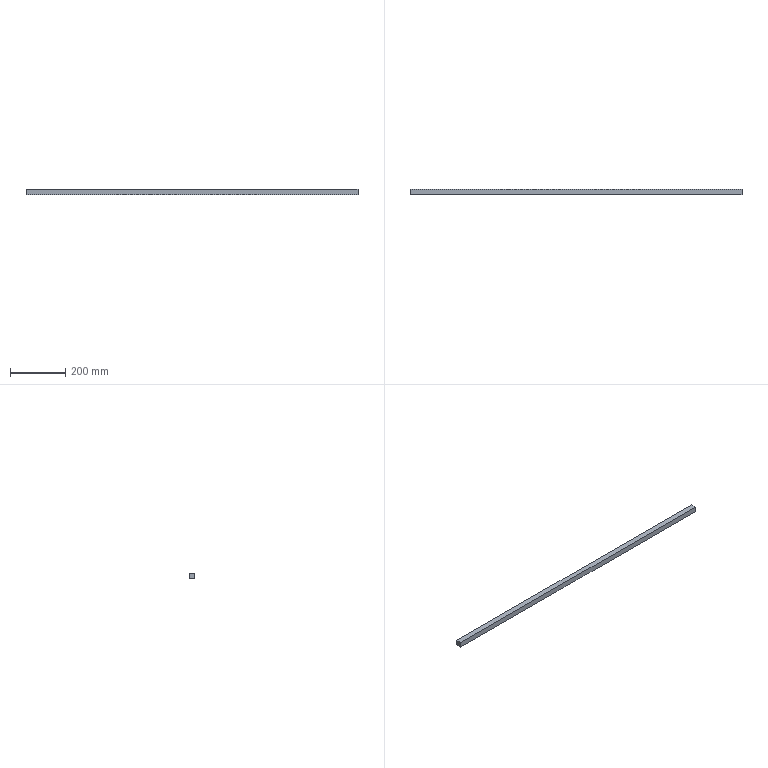Component | SolidWorks | GuideRailSchematic-2 | 1 solid | 6 faces | box 1200 x 20 x 20 mm | volume 480000 mm3 | plane 6
build123d program:
from build123d import *

# Parameters (mm, degrees)
SKETCH1_W           = 20
SKETCH1_H           = 20
BOSS_EXTRUDE1_DEPTH = 600


with BuildPart() as part:
    # Sketch1 → Boss-Extrude1 (new, symmetric)
    with BuildSketch(Plane.XY):
        Rectangle(SKETCH1_W, SKETCH1_H)
    extrude(amount=BOSS_EXTRUDE1_DEPTH, both=True)


solid = part.part

# Placed as in the assembly
solid = solid.moved(Location((-60.068, -205.375, 1233.05), (0, 90, 0)))
STEP:
#1=CARTESIAN_POINT('',(21.257,-7.692,48.152));
#2=VERTEX_POINT('',#1);
#3=CARTESIAN_POINT('',(21.257,-8.479,48.152));
#4=VERTEX_POINT('',#3);
#5=CARTESIAN_POINT('',(21.257,-8.479,48.152));
#6=DIRECTION('',(0.,-1.,-0.));
#7=VECTOR('',#6,39.37);
#8=LINE('',#5,#7);
#9=EDGE_CURVE('',#2,#4,#8,.T.);
#10=ORIENTED_EDGE('',*,*,#9,.T.);
#11=CARTESIAN_POINT('',(-25.987,-8.479,48.152));
#12=VERTEX_POINT('',#11);
#13=CARTESIAN_POINT('',(-25.987,-8.479,48.152));
#14=DIRECTION('',(1.,0.,-0.));
#15=VECTOR('',#14,39.37);
#16=LINE('',#13,#15);
#17=EDGE_CURVE('',#12,#4,#16,.T.);
#18=ORIENTED_EDGE('',*,*,#17,.F.);
#19=CARTESIAN_POINT('',(-25.987,-7.692,48.152));
#20=VERTEX_POINT('',#19);
#21=CARTESIAN_POINT('',(-25.987,-8.479,48.152));
#22=DIRECTION('',(0.,-1.,-0.));
#23=VECTOR('',#22,39.37);
#24=LINE('',#21,#23);
#25=EDGE_CURVE('',#20,#12,#24,.T.);
#26=ORIENTED_EDGE('',*,*,#25,.F.);
#27=CARTESIAN_POINT('',(-25.987,-7.692,48.152));
#28=DIRECTION('',(1.,0.,-0.));
#29=VECTOR('',#28,39.37);
#30=LINE('',#27,#29);
#31=EDGE_CURVE('',#20,#2,#30,.T.);
#32=ORIENTED_EDGE('',*,*,#31,.T.);
#33=EDGE_LOOP('',(#10,#18,#26,#32));
#34=FACE_OUTER_BOUND('',#33,.T.);
#35=CARTESIAN_POINT('',(-25.987,-8.479,48.152));
#36=DIRECTION('',(0.,-0.,1.));
#37=DIRECTION('',(1.,0.,-0.));
#38=AXIS2_PLACEMENT_3D('',#35,#36,#37);
#39=PLANE('',#38);
#40=ADVANCED_FACE('',(#34),#39,.F.);
#41=CARTESIAN_POINT('',(21.257,-8.479,48.939));
#42=VERTEX_POINT('',#41);
#43=CARTESIAN_POINT('',(21.257,-8.479,48.939));
#44=DIRECTION('',(0.,-0.,1.));
#45=VECTOR('',#44,39.37);
#46=LINE('',#43,#45);
#47=EDGE_CURVE('',#4,#42,#46,.T.);
#48=ORIENTED_EDGE('',*,*,#47,.T.);
#49=CARTESIAN_POINT('',(-25.987,-8.479,48.939));
#50=VERTEX_POINT('',#49);
#51=CARTESIAN_POINT('',(-25.987,-8.479,48.939));
#52=DIRECTION('',(1.,0.,-0.));
#53=VECTOR('',#52,39.37);
#54=LINE('',#51,#53);
#55=EDGE_CURVE('',#50,#42,#54,.T.);
#56=ORIENTED_EDGE('',*,*,#55,.F.);
#57=CARTESIAN_POINT('',(-25.987,-8.479,48.939));
#58=DIRECTION('',(0.,-0.,1.));
#59=VECTOR('',#58,39.37);
#60=LINE('',#57,#59);
#61=EDGE_CURVE('',#12,#50,#60,.T.);
#62=ORIENTED_EDGE('',*,*,#61,.F.);
#63=ORIENTED_EDGE('',*,*,#17,.T.);
#64=EDGE_LOOP('',(#48,#56,#62,#63));
#65=FACE_OUTER_BOUND('',#64,.T.);
#66=CARTESIAN_POINT('',(-25.987,-8.479,48.939));
#67=DIRECTION('',(-0.,1.,0.));
#68=DIRECTION('',(-0.,0.,-1.));
#69=AXIS2_PLACEMENT_3D('',#66,#67,#68);
#70=PLANE('',#69);
#71=ADVANCED_FACE('',(#65),#70,.F.);
#72=CARTESIAN_POINT('',(21.257,-7.692,48.939));
#73=VERTEX_POINT('',#72);
#74=CARTESIAN_POINT('',(21.257,-8.479,48.939));
#75=DIRECTION('',(-0.,1.,0.));
#76=VECTOR('',#75,39.37);
#77=LINE('',#74,#76);
#78=EDGE_CURVE('',#42,#73,#77,.T.);
#79=ORIENTED_EDGE('',*,*,#78,.T.);
#80=CARTESIAN_POINT('',(-25.987,-7.692,48.939));
#81=VERTEX_POINT('',#80);
#82=CARTESIAN_POINT('',(-25.987,-7.692,48.939));
#83=DIRECTION('',(1.,0.,-0.));
#84=VECTOR('',#83,39.37);
#85=LINE('',#82,#84);
#86=EDGE_CURVE('',#81,#73,#85,.T.);
#87=ORIENTED_EDGE('',*,*,#86,.F.);
#88=CARTESIAN_POINT('',(-25.987,-8.479,48.939));
#89=DIRECTION('',(-0.,1.,0.));
#90=VECTOR('',#89,39.37);
#91=LINE('',#88,#90);
#92=EDGE_CURVE('',#50,#81,#91,.T.);
#93=ORIENTED_EDGE('',*,*,#92,.F.);
#94=ORIENTED_EDGE('',*,*,#55,.T.);
#95=EDGE_LOOP('',(#79,#87,#93,#94));
#96=FACE_OUTER_BOUND('',#95,.T.);
#97=CARTESIAN_POINT('',(-25.987,-8.479,48.939));
#98=DIRECTION('',(-0.,0.,-1.));
#99=DIRECTION('',(-1.,-0.,0.));
#100=AXIS2_PLACEMENT_3D('',#97,#98,#99);
#101=PLANE('',#100);
#102=ADVANCED_FACE('',(#96),#101,.F.);
#103=CARTESIAN_POINT('',(21.257,-7.692,48.939));
#104=DIRECTION('',(-0.,0.,-1.));
#105=VECTOR('',#104,39.37);
#106=LINE('',#103,#105);
#107=EDGE_CURVE('',#73,#2,#106,.T.);
#108=ORIENTED_EDGE('',*,*,#107,.T.);
#109=ORIENTED_EDGE('',*,*,#31,.F.);
#110=CARTESIAN_POINT('',(-25.987,-7.692,48.939));
#111=DIRECTION('',(-0.,0.,-1.));
#112=VECTOR('',#111,39.37);
#113=LINE('',#110,#112);
#114=EDGE_CURVE('',#81,#20,#113,.T.);
#115=ORIENTED_EDGE('',*,*,#114,.F.);
#116=ORIENTED_EDGE('',*,*,#86,.T.);
#117=EDGE_LOOP('',(#108,#109,#115,#116));
#118=FACE_OUTER_BOUND('',#117,.T.);
#119=CARTESIAN_POINT('',(-25.987,-7.692,48.939));
#120=DIRECTION('',(0.,-1.,-0.));
#121=DIRECTION('',(0.,-0.,1.));
#122=AXIS2_PLACEMENT_3D('',#119,#120,#121);
#123=PLANE('',#122);
#124=ADVANCED_FACE('',(#118),#123,.F.);
#125=ORIENTED_EDGE('',*,*,#25,.T.);
#126=ORIENTED_EDGE('',*,*,#61,.T.);
#127=ORIENTED_EDGE('',*,*,#92,.T.);
#128=ORIENTED_EDGE('',*,*,#114,.T.);
#129=EDGE_LOOP('',(#125,#126,#127,#128));
#130=FACE_OUTER_BOUND('',#129,.T.);
#131=CARTESIAN_POINT('',(-25.987,-8.086,48.545));
#132=DIRECTION('',(-1.,-0.,0.));
#133=DIRECTION('',(0.,-0.,1.));
#134=AXIS2_PLACEMENT_3D('',#131,#132,#133);
#135=PLANE('',#134);
#136=ADVANCED_FACE('',(#130),#135,.T.);
#137=ORIENTED_EDGE('',*,*,#9,.F.);
#138=ORIENTED_EDGE('',*,*,#107,.F.);
#139=ORIENTED_EDGE('',*,*,#78,.F.);
#140=ORIENTED_EDGE('',*,*,#47,.F.);
#141=EDGE_LOOP('',(#137,#138,#139,#140));
#142=FACE_OUTER_BOUND('',#141,.T.);
#143=CARTESIAN_POINT('',(21.257,-8.086,48.545));
#144=DIRECTION('',(-1.,-0.,0.));
#145=DIRECTION('',(0.,-0.,1.));
#146=AXIS2_PLACEMENT_3D('',#143,#144,#145);
#147=PLANE('',#146);
#148=ADVANCED_FACE('',(#142),#147,.F.);
#149=CLOSED_SHELL('',(#40,#71,#102,#124,#136,#148));
#150=MANIFOLD_SOLID_BREP('',#149);
#151=CARTESIAN_POINT('',(0.,0.,0.));
#152=DIRECTION('',(0.,0.,1.));
#153=DIRECTION('',(1.,0.,0.));
#154=AXIS2_PLACEMENT_3D('',#151,#152,#153);
#155=(LENGTH_UNIT()NAMED_UNIT(*)SI_UNIT($,.METRE.));
#156=LENGTH_MEASURE_WITH_UNIT(LENGTH_MEASURE(0.0254),#155);
#157=DIMENSIONAL_EXPONENTS(1.,0.,0.,0.,0.,0.,0.);
#158=(CONVERSION_BASED_UNIT('',#156)LENGTH_UNIT()NAMED_UNIT(#157));
#159=UNCERTAINTY_MEASURE_WITH_UNIT(LENGTH_MEASURE(0.00001),#158,'','');
#160=(NAMED_UNIT(*)PLANE_ANGLE_UNIT()SI_UNIT($,.RADIAN.));
#161=(NAMED_UNIT(*)SI_UNIT($,.STERADIAN.)SOLID_ANGLE_UNIT());
#162=(GEOMETRIC_REPRESENTATION_CONTEXT(3)GLOBAL_UNCERTAINTY_ASSIGNED_CONTEXT((#159))GLOBAL_UNIT_ASSIGNED_CONTEXT((#158,#160,#161))REPRESENTATION_CONTEXT('',''));
#163=ADVANCED_BREP_SHAPE_REPRESENTATION('',(#150,#154),#162);
#164=COLOUR_RGB('',0.7922,0.8196,0.9333);
#165=FILL_AREA_STYLE_COLOUR('',#164);
#166=FILL_AREA_STYLE('',(#165));
#167=SURFACE_STYLE_FILL_AREA(#166);
#168=SURFACE_SIDE_STYLE('',(#167));
#169=SURFACE_STYLE_USAGE(.BOTH.,#168);
#170=PRESENTATION_STYLE_ASSIGNMENT((#169));
#171=STYLED_ITEM('',(#170),#150);
#172=PRESENTATION_LAYER_ASSIGNMENT('','',(#171));
#173=(LENGTH_UNIT()NAMED_UNIT(*)SI_UNIT($,.METRE.));
#174=LENGTH_MEASURE_WITH_UNIT(LENGTH_MEASURE(0.0254),#173);
#175=DIMENSIONAL_EXPONENTS(1.,0.,0.,0.,0.,0.,0.);
#176=(CONVERSION_BASED_UNIT('',#174)LENGTH_UNIT()NAMED_UNIT(#175));
#177=UNCERTAINTY_MEASURE_WITH_UNIT(LENGTH_MEASURE(0.00001),#176,'','');
#178=(NAMED_UNIT(*)PLANE_ANGLE_UNIT()SI_UNIT($,.RADIAN.));
#179=(NAMED_UNIT(*)SI_UNIT($,.STERADIAN.)SOLID_ANGLE_UNIT());
#180=(GEOMETRIC_REPRESENTATION_CONTEXT(3)GLOBAL_UNCERTAINTY_ASSIGNED_CONTEXT((#177))GLOBAL_UNIT_ASSIGNED_CONTEXT((#176,#178,#179))REPRESENTATION_CONTEXT('',''));
#181=MECHANICAL_DESIGN_GEOMETRIC_PRESENTATION_REPRESENTATION('',(#171),#180);